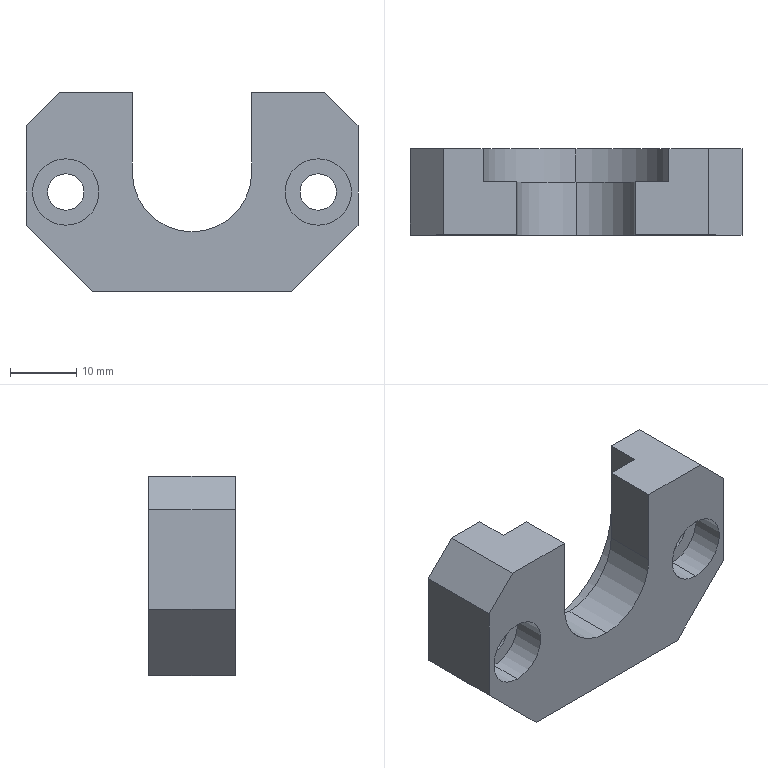Component | SolidWorks | F12529-M5112-1 | 1 solid | 30 faces | box 50 x 13 x 30 mm | volume 10744 mm3 | plane 18 | cylinder 12 | commonest cylinder face diameters 10 x4 5.5 x4 28 x2 18 x2
build123d program:
from build123d import *

# Parameters (mm, degrees)
SKETCH1_W                                            = 50
SKETCH1_H                                            = 30
BOSS_EXTRUDE1_DEPTH                                  = 13
CUT_EXTRUDE2_DEPTH                                   = 32.922
CUT_EXTRUDE3_DEPTH                                   = 5
M5_HEX_SOCKET_HEAD_CAP_SCREW_COUNTERBORE_D           = 5.5
M5_HEX_SOCKET_HEAD_CAP_SCREW_COUNTERBORE_CBORE_D     = 10
M5_HEX_SOCKET_HEAD_CAP_SCREW_COUNTERBORE_CBORE_DEPTH = 5
CHAMFER1_SIZE                                        = 5
CHAMFER2_SIZE                                        = 10


with BuildPart() as part:
    # Sketch1 → Boss-Extrude1 (new body)
    with BuildSketch(Plane(origin=(0, 0, 0), x_dir=(1, 0, 0), z_dir=(0, 1, 0))):
        Rectangle(SKETCH1_W, SKETCH1_H)
    extrude(amount=BOSS_EXTRUDE1_DEPTH)

    # Sketch2 → Cut-Extrude2 (cut, through all)
    with BuildSketch(Plane(origin=(0, 13, 0), x_dir=(1, 0, 0), z_dir=(0, 1, 0))):
        with BuildLine():
            Line((-9, 15), (9, 15))
            Line((9, 15), (9, 3))
            ThreePointArc((9, 3), (0, -6), (-9, 3))
            Line((-9, 3), (-9, 15))
        make_face()
    extrude(amount=-CUT_EXTRUDE2_DEPTH, mode=Mode.SUBTRACT)

    # Sketch3 → Cut-Extrude3 (cut)
    with BuildSketch(Plane(origin=(0, 13, 0), x_dir=(1, 0, 0), z_dir=(0, 1, 0))):
        with BuildLine():
            Line((-14, 15), (14, 15))
            Line((14, 15), (14, 3))
            ThreePointArc((14, 3), (0, -11), (-14, 3))
            Line((-14, 3), (-14, 15))
        make_face()
    extrude(amount=-CUT_EXTRUDE3_DEPTH, mode=Mode.SUBTRACT)

    # M5 Hex Socket Head Cap Screw Counterbore (through all)
    with Locations(Plane.XZ):
        with Locations((19, 0), (-19, 0)):
            CounterBoreHole(M5_HEX_SOCKET_HEAD_CAP_SCREW_COUNTERBORE_D / 2, M5_HEX_SOCKET_HEAD_CAP_SCREW_COUNTERBORE_CBORE_D / 2, M5_HEX_SOCKET_HEAD_CAP_SCREW_COUNTERBORE_CBORE_DEPTH)

    # Chamfer1
    chamfer1_edges = [part.edges().sort_by_distance(p)[0] for p in [
        (-25, 6.5, -15),
        (25, 6.5, -15),
    ]]
    chamfer(chamfer1_edges, length=CHAMFER1_SIZE)

    # Chamfer2
    chamfer2_edges = [part.edges().sort_by_distance(p)[0] for p in [
        (25, 6.5, 15),
        (-25, 6.5, 15),
    ]]
    chamfer(chamfer2_edges, length=CHAMFER2_SIZE)


solid = part.part

# Placed as in the assembly
solid = solid.moved(Location((0, 108, -3), (-180, 0, 180)))
STEP:
#1=CARTESIAN_POINT('',(-0.748,4.449,-0.315));
#2=VERTEX_POINT('',#1);
#3=CARTESIAN_POINT('',(-0.748,4.449,0.07874));
#4=VERTEX_POINT('',#3);
#5=CARTESIAN_POINT('',(-0.748,4.449,-0.1181));
#6=DIRECTION('',(-0.,-1.,-0.));
#7=DIRECTION('',(0.,0.,1.));
#8=AXIS2_PLACEMENT_3D('',#5,#6,#7);
#9=CIRCLE('',#8,0.1969);
#10=EDGE_CURVE('',#2,#4,#9,.T.);
#11=ORIENTED_EDGE('',*,*,#10,.F.);
#12=CARTESIAN_POINT('',(-0.748,4.252,-0.315));
#13=VERTEX_POINT('',#12);
#14=CARTESIAN_POINT('',(-0.748,4.252,-0.315));
#15=DIRECTION('',(-0.,-1.,-0.));
#16=VECTOR('',#15,39.37);
#17=LINE('',#14,#16);
#18=EDGE_CURVE('',#2,#13,#17,.T.);
#19=ORIENTED_EDGE('',*,*,#18,.T.);
#20=CARTESIAN_POINT('',(-0.748,4.252,0.07874));
#21=VERTEX_POINT('',#20);
#22=CARTESIAN_POINT('',(-0.748,4.252,-0.1181));
#23=DIRECTION('',(-0.,-1.,-0.));
#24=DIRECTION('',(0.,0.,1.));
#25=AXIS2_PLACEMENT_3D('',#22,#23,#24);
#26=CIRCLE('',#25,0.1969);
#27=EDGE_CURVE('',#13,#21,#26,.T.);
#28=ORIENTED_EDGE('',*,*,#27,.T.);
#29=CARTESIAN_POINT('',(-0.748,4.252,0.07874));
#30=DIRECTION('',(-0.,-1.,-0.));
#31=VECTOR('',#30,39.37);
#32=LINE('',#29,#31);
#33=EDGE_CURVE('',#4,#21,#32,.T.);
#34=ORIENTED_EDGE('',*,*,#33,.F.);
#35=EDGE_LOOP('',(#11,#19,#28,#34));
#36=FACE_OUTER_BOUND('',#35,.T.);
#37=CARTESIAN_POINT('',(-0.748,4.252,-0.1181));
#38=DIRECTION('',(-0.,-1.,-0.));
#39=DIRECTION('',(0.,0.,1.));
#40=AXIS2_PLACEMENT_3D('',#37,#38,#39);
#41=CYLINDRICAL_SURFACE('',#40,0.1969);
#42=ADVANCED_FACE('',(#36),#41,.F.);
#43=CARTESIAN_POINT('',(-0.748,4.764,-0.2264));
#44=VERTEX_POINT('',#43);
#45=CARTESIAN_POINT('',(-0.748,4.764,-0.009843));
#46=VERTEX_POINT('',#45);
#47=CARTESIAN_POINT('',(-0.748,4.764,-0.1181));
#48=DIRECTION('',(-0.,-1.,-0.));
#49=DIRECTION('',(0.,0.,1.));
#50=AXIS2_PLACEMENT_3D('',#47,#48,#49);
#51=CIRCLE('',#50,0.1083);
#52=EDGE_CURVE('',#44,#46,#51,.T.);
#53=ORIENTED_EDGE('',*,*,#52,.F.);
#54=CARTESIAN_POINT('',(-0.748,4.449,-0.2264));
#55=VERTEX_POINT('',#54);
#56=CARTESIAN_POINT('',(-0.748,4.252,-0.2264));
#57=DIRECTION('',(-0.,-1.,-0.));
#58=VECTOR('',#57,39.37);
#59=LINE('',#56,#58);
#60=EDGE_CURVE('',#44,#55,#59,.T.);
#61=ORIENTED_EDGE('',*,*,#60,.T.);
#62=CARTESIAN_POINT('',(-0.748,4.449,-0.009843));
#63=VERTEX_POINT('',#62);
#64=CARTESIAN_POINT('',(-0.748,4.449,-0.1181));
#65=DIRECTION('',(-0.,-1.,-0.));
#66=DIRECTION('',(0.,0.,1.));
#67=AXIS2_PLACEMENT_3D('',#64,#65,#66);
#68=CIRCLE('',#67,0.1083);
#69=EDGE_CURVE('',#55,#63,#68,.T.);
#70=ORIENTED_EDGE('',*,*,#69,.T.);
#71=CARTESIAN_POINT('',(-0.748,4.252,-0.009843));
#72=DIRECTION('',(-0.,-1.,-0.));
#73=VECTOR('',#72,39.37);
#74=LINE('',#71,#73);
#75=EDGE_CURVE('',#46,#63,#74,.T.);
#76=ORIENTED_EDGE('',*,*,#75,.F.);
#77=EDGE_LOOP('',(#53,#61,#70,#76));
#78=FACE_OUTER_BOUND('',#77,.T.);
#79=CARTESIAN_POINT('',(-0.748,4.252,-0.1181));
#80=DIRECTION('',(-0.,-1.,-0.));
#81=DIRECTION('',(0.,0.,1.));
#82=AXIS2_PLACEMENT_3D('',#79,#80,#81);
#83=CYLINDRICAL_SURFACE('',#82,0.1083);
#84=ADVANCED_FACE('',(#78),#83,.F.);
#85=CARTESIAN_POINT('',(0.748,4.449,-0.315));
#86=VERTEX_POINT('',#85);
#87=CARTESIAN_POINT('',(0.748,4.449,0.07874));
#88=VERTEX_POINT('',#87);
#89=CARTESIAN_POINT('',(0.748,4.449,-0.1181));
#90=DIRECTION('',(-0.,-1.,-0.));
#91=DIRECTION('',(0.,0.,1.));
#92=AXIS2_PLACEMENT_3D('',#89,#90,#91);
#93=CIRCLE('',#92,0.1969);
#94=EDGE_CURVE('',#86,#88,#93,.T.);
#95=ORIENTED_EDGE('',*,*,#94,.F.);
#96=CARTESIAN_POINT('',(0.748,4.252,-0.315));
#97=VERTEX_POINT('',#96);
#98=CARTESIAN_POINT('',(0.748,4.252,-0.315));
#99=DIRECTION('',(-0.,-1.,-0.));
#100=VECTOR('',#99,39.37);
#101=LINE('',#98,#100);
#102=EDGE_CURVE('',#86,#97,#101,.T.);
#103=ORIENTED_EDGE('',*,*,#102,.T.);
#104=CARTESIAN_POINT('',(0.748,4.252,0.07874));
#105=VERTEX_POINT('',#104);
#106=CARTESIAN_POINT('',(0.748,4.252,-0.1181));
#107=DIRECTION('',(-0.,-1.,-0.));
#108=DIRECTION('',(0.,0.,1.));
#109=AXIS2_PLACEMENT_3D('',#106,#107,#108);
#110=CIRCLE('',#109,0.1969);
#111=EDGE_CURVE('',#97,#105,#110,.T.);
#112=ORIENTED_EDGE('',*,*,#111,.T.);
#113=CARTESIAN_POINT('',(0.748,4.252,0.07874));
#114=DIRECTION('',(-0.,-1.,-0.));
#115=VECTOR('',#114,39.37);
#116=LINE('',#113,#115);
#117=EDGE_CURVE('',#88,#105,#116,.T.);
#118=ORIENTED_EDGE('',*,*,#117,.F.);
#119=EDGE_LOOP('',(#95,#103,#112,#118));
#120=FACE_OUTER_BOUND('',#119,.T.);
#121=CARTESIAN_POINT('',(0.748,4.252,-0.1181));
#122=DIRECTION('',(-0.,-1.,-0.));
#123=DIRECTION('',(0.,0.,1.));
#124=AXIS2_PLACEMENT_3D('',#121,#122,#123);
#125=CYLINDRICAL_SURFACE('',#124,0.1969);
#126=ADVANCED_FACE('',(#120),#125,.F.);
#127=CARTESIAN_POINT('',(0.748,4.764,-0.2264));
#128=VERTEX_POINT('',#127);
#129=CARTESIAN_POINT('',(0.748,4.764,-0.009843));
#130=VERTEX_POINT('',#129);
#131=CARTESIAN_POINT('',(0.748,4.764,-0.1181));
#132=DIRECTION('',(-0.,-1.,-0.));
#133=DIRECTION('',(0.,0.,1.));
#134=AXIS2_PLACEMENT_3D('',#131,#132,#133);
#135=CIRCLE('',#134,0.1083);
#136=EDGE_CURVE('',#128,#130,#135,.T.);
#137=ORIENTED_EDGE('',*,*,#136,.F.);
#138=CARTESIAN_POINT('',(0.748,4.449,-0.2264));
#139=VERTEX_POINT('',#138);
#140=CARTESIAN_POINT('',(0.748,4.252,-0.2264));
#141=DIRECTION('',(-0.,-1.,-0.));
#142=VECTOR('',#141,39.37);
#143=LINE('',#140,#142);
#144=EDGE_CURVE('',#128,#139,#143,.T.);
#145=ORIENTED_EDGE('',*,*,#144,.T.);
#146=CARTESIAN_POINT('',(0.748,4.449,-0.009843));
#147=VERTEX_POINT('',#146);
#148=CARTESIAN_POINT('',(0.748,4.449,-0.1181));
#149=DIRECTION('',(-0.,-1.,-0.));
#150=DIRECTION('',(0.,0.,1.));
#151=AXIS2_PLACEMENT_3D('',#148,#149,#150);
#152=CIRCLE('',#151,0.1083);
#153=EDGE_CURVE('',#139,#147,#152,.T.);
#154=ORIENTED_EDGE('',*,*,#153,.T.);
#155=CARTESIAN_POINT('',(0.748,4.252,-0.009843));
#156=DIRECTION('',(-0.,-1.,-0.));
#157=VECTOR('',#156,39.37);
#158=LINE('',#155,#157);
#159=EDGE_CURVE('',#130,#147,#158,.T.);
#160=ORIENTED_EDGE('',*,*,#159,.F.);
#161=EDGE_LOOP('',(#137,#145,#154,#160));
#162=FACE_OUTER_BOUND('',#161,.T.);
#163=CARTESIAN_POINT('',(0.748,4.252,-0.1181));
#164=DIRECTION('',(-0.,-1.,-0.));
#165=DIRECTION('',(0.,0.,1.));
#166=AXIS2_PLACEMENT_3D('',#163,#164,#165);
#167=CYLINDRICAL_SURFACE('',#166,0.1083);
#168=ADVANCED_FACE('',(#162),#167,.F.);
#169=CARTESIAN_POINT('',(0.,4.567,-0.5512));
#170=VERTEX_POINT('',#169);
#171=CARTESIAN_POINT('',(-0.5512,4.567,0.));
#172=VERTEX_POINT('',#171);
#173=CARTESIAN_POINT('',(0.,4.567,0.));
#174=DIRECTION('',(0.,1.,0.));
#175=DIRECTION('',(-0.,0.,1.));
#176=AXIS2_PLACEMENT_3D('',#173,#174,#175);
#177=CIRCLE('',#176,0.5512);
#178=EDGE_CURVE('',#170,#172,#177,.T.);
#179=ORIENTED_EDGE('',*,*,#178,.F.);
#180=CARTESIAN_POINT('',(0.,4.764,-0.5512));
#181=VERTEX_POINT('',#180);
#182=CARTESIAN_POINT('',(0.,4.567,-0.5512));
#183=DIRECTION('',(0.,1.,0.));
#184=VECTOR('',#183,39.37);
#185=LINE('',#182,#184);
#186=EDGE_CURVE('',#170,#181,#185,.T.);
#187=ORIENTED_EDGE('',*,*,#186,.T.);
#188=CARTESIAN_POINT('',(-0.5512,4.764,0.));
#189=VERTEX_POINT('',#188);
#190=CARTESIAN_POINT('',(0.,4.764,0.));
#191=DIRECTION('',(0.,1.,0.));
#192=DIRECTION('',(-0.,0.,1.));
#193=AXIS2_PLACEMENT_3D('',#190,#191,#192);
#194=CIRCLE('',#193,0.5512);
#195=EDGE_CURVE('',#181,#189,#194,.T.);
#196=ORIENTED_EDGE('',*,*,#195,.T.);
#197=CARTESIAN_POINT('',(-0.5512,4.567,0.));
#198=DIRECTION('',(0.,1.,0.));
#199=VECTOR('',#198,39.37);
#200=LINE('',#197,#199);
#201=EDGE_CURVE('',#172,#189,#200,.T.);
#202=ORIENTED_EDGE('',*,*,#201,.F.);
#203=EDGE_LOOP('',(#179,#187,#196,#202));
#204=FACE_OUTER_BOUND('',#203,.T.);
#205=CARTESIAN_POINT('',(0.,4.567,0.));
#206=DIRECTION('',(0.,1.,0.));
#207=DIRECTION('',(0.,0.,-1.));
#208=AXIS2_PLACEMENT_3D('',#205,#206,#207);
#209=CYLINDRICAL_SURFACE('',#208,0.5512);
#210=ADVANCED_FACE('',(#204),#209,.F.);
#211=CARTESIAN_POINT('',(0.,4.252,-0.3543));
#212=VERTEX_POINT('',#211);
#213=CARTESIAN_POINT('',(-0.3543,4.252,0.));
#214=VERTEX_POINT('',#213);
#215=CARTESIAN_POINT('',(0.,4.252,0.));
#216=DIRECTION('',(0.,1.,0.));
#217=DIRECTION('',(-0.,0.,1.));
#218=AXIS2_PLACEMENT_3D('',#215,#216,#217);
#219=CIRCLE('',#218,0.3543);
#220=EDGE_CURVE('',#212,#214,#219,.T.);
#221=ORIENTED_EDGE('',*,*,#220,.F.);
#222=CARTESIAN_POINT('',(0.,4.567,-0.3543));
#223=VERTEX_POINT('',#222);
#224=CARTESIAN_POINT('',(0.,4.252,-0.3543));
#225=DIRECTION('',(0.,1.,0.));
#226=VECTOR('',#225,39.37);
#227=LINE('',#224,#226);
#228=EDGE_CURVE('',#212,#223,#227,.T.);
#229=ORIENTED_EDGE('',*,*,#228,.T.);
#230=CARTESIAN_POINT('',(-0.3543,4.567,0.));
#231=VERTEX_POINT('',#230);
#232=CARTESIAN_POINT('',(0.,4.567,0.));
#233=DIRECTION('',(0.,1.,0.));
#234=DIRECTION('',(-0.,0.,1.));
#235=AXIS2_PLACEMENT_3D('',#232,#233,#234);
#236=CIRCLE('',#235,0.3543);
#237=EDGE_CURVE('',#223,#231,#236,.T.);
#238=ORIENTED_EDGE('',*,*,#237,.T.);
#239=CARTESIAN_POINT('',(-0.3543,4.252,0.));
#240=DIRECTION('',(0.,1.,0.));
#241=VECTOR('',#240,39.37);
#242=LINE('',#239,#241);
#243=EDGE_CURVE('',#214,#231,#242,.T.);
#244=ORIENTED_EDGE('',*,*,#243,.F.);
#245=EDGE_LOOP('',(#221,#229,#238,#244));
#246=FACE_OUTER_BOUND('',#245,.T.);
#247=CARTESIAN_POINT('',(0.,4.252,0.));
#248=DIRECTION('',(0.,1.,0.));
#249=DIRECTION('',(0.,0.,-1.));
#250=AXIS2_PLACEMENT_3D('',#247,#248,#249);
#251=CYLINDRICAL_SURFACE('',#250,0.3543);
#252=ADVANCED_FACE('',(#246),#251,.F.);
#253=CARTESIAN_POINT('',(0.3543,4.252,0.4724));
#254=VERTEX_POINT('',#253);
#255=CARTESIAN_POINT('',(0.7874,4.252,0.4724));
#256=VERTEX_POINT('',#255);
#257=CARTESIAN_POINT('',(0.9843,4.252,0.4724));
#258=DIRECTION('',(1.,-0.,0.));
#259=VECTOR('',#258,39.37);
#260=LINE('',#257,#259);
#261=EDGE_CURVE('',#254,#256,#260,.T.);
#262=ORIENTED_EDGE('',*,*,#261,.T.);
#263=CARTESIAN_POINT('',(0.7874,4.764,0.4724));
#264=VERTEX_POINT('',#263);
#265=CARTESIAN_POINT('',(0.7874,4.764,0.4724));
#266=DIRECTION('',(0.,1.,0.));
#267=VECTOR('',#266,39.37);
#268=LINE('',#265,#267);
#269=EDGE_CURVE('',#256,#264,#268,.T.);
#270=ORIENTED_EDGE('',*,*,#269,.T.);
#271=CARTESIAN_POINT('',(0.5512,4.764,0.4724));
#272=VERTEX_POINT('',#271);
#273=CARTESIAN_POINT('',(0.9843,4.764,0.4724));
#274=DIRECTION('',(1.,-0.,0.));
#275=VECTOR('',#274,39.37);
#276=LINE('',#273,#275);
#277=EDGE_CURVE('',#272,#264,#276,.T.);
#278=ORIENTED_EDGE('',*,*,#277,.F.);
#279=CARTESIAN_POINT('',(0.5512,4.567,0.4724));
#280=VERTEX_POINT('',#279);
#281=CARTESIAN_POINT('',(0.5512,4.567,0.4724));
#282=DIRECTION('',(0.,1.,0.));
#283=VECTOR('',#282,39.37);
#284=LINE('',#281,#283);
#285=EDGE_CURVE('',#280,#272,#284,.T.);
#286=ORIENTED_EDGE('',*,*,#285,.F.);
#287=CARTESIAN_POINT('',(0.3543,4.567,0.4724));
#288=VERTEX_POINT('',#287);
#289=CARTESIAN_POINT('',(0.5512,4.567,0.4724));
#290=DIRECTION('',(1.,-0.,0.));
#291=VECTOR('',#290,39.37);
#292=LINE('',#289,#291);
#293=EDGE_CURVE('',#288,#280,#292,.T.);
#294=ORIENTED_EDGE('',*,*,#293,.F.);
#295=CARTESIAN_POINT('',(0.3543,4.252,0.4724));
#296=DIRECTION('',(0.,1.,0.));
#297=VECTOR('',#296,39.37);
#298=LINE('',#295,#297);
#299=EDGE_CURVE('',#254,#288,#298,.T.);
#300=ORIENTED_EDGE('',*,*,#299,.F.);
#301=EDGE_LOOP('',(#262,#270,#278,#286,#294,#300));
#302=FACE_OUTER_BOUND('',#301,.T.);
#303=CARTESIAN_POINT('',(0.9843,4.764,0.4724));
#304=DIRECTION('',(0.,0.,-1.));
#305=DIRECTION('',(-1.,0.,-0.));
#306=AXIS2_PLACEMENT_3D('',#303,#304,#305);
#307=PLANE('',#306);
#308=ADVANCED_FACE('',(#302),#307,.F.);
#309=CARTESIAN_POINT('',(0.9843,4.252,0.2756));
#310=VERTEX_POINT('',#309);
#311=CARTESIAN_POINT('',(0.9843,4.252,-0.315));
#312=VERTEX_POINT('',#311);
#313=CARTESIAN_POINT('',(0.9843,4.252,0.4724));
#314=DIRECTION('',(-0.,0.,-1.));
#315=VECTOR('',#314,39.37);
#316=LINE('',#313,#315);
#317=EDGE_CURVE('',#310,#312,#316,.T.);
#318=ORIENTED_EDGE('',*,*,#317,.T.);
#319=CARTESIAN_POINT('',(0.9843,4.764,-0.315));
#320=VERTEX_POINT('',#319);
#321=CARTESIAN_POINT('',(0.9843,4.764,-0.315));
#322=DIRECTION('',(0.,1.,0.));
#323=VECTOR('',#322,39.37);
#324=LINE('',#321,#323);
#325=EDGE_CURVE('',#312,#320,#324,.T.);
#326=ORIENTED_EDGE('',*,*,#325,.T.);
#327=CARTESIAN_POINT('',(0.9843,4.764,0.2756));
#328=VERTEX_POINT('',#327);
#329=CARTESIAN_POINT('',(0.9843,4.764,0.4724));
#330=DIRECTION('',(-0.,0.,-1.));
#331=VECTOR('',#330,39.37);
#332=LINE('',#329,#331);
#333=EDGE_CURVE('',#328,#320,#332,.T.);
#334=ORIENTED_EDGE('',*,*,#333,.F.);
#335=CARTESIAN_POINT('',(0.9843,4.764,0.2756));
#336=DIRECTION('',(-0.,-1.,-0.));
#337=VECTOR('',#336,39.37);
#338=LINE('',#335,#337);
#339=EDGE_CURVE('',#328,#310,#338,.T.);
#340=ORIENTED_EDGE('',*,*,#339,.T.);
#341=EDGE_LOOP('',(#318,#326,#334,#340));
#342=FACE_OUTER_BOUND('',#341,.T.);
#343=CARTESIAN_POINT('',(0.9843,4.764,0.4724));
#344=DIRECTION('',(-1.,0.,0.));
#345=DIRECTION('',(0.,-0.,1.));
#346=AXIS2_PLACEMENT_3D('',#343,#344,#345);
#347=PLANE('',#346);
#348=ADVANCED_FACE('',(#342),#347,.F.);
#349=CARTESIAN_POINT('',(0.5906,4.252,-0.7087));
#350=VERTEX_POINT('',#349);
#351=CARTESIAN_POINT('',(-0.5906,4.252,-0.7087));
#352=VERTEX_POINT('',#351);
#353=CARTESIAN_POINT('',(0.9843,4.252,-0.7087));
#354=DIRECTION('',(-1.,0.,-0.));
#355=VECTOR('',#354,39.37);
#356=LINE('',#353,#355);
#357=EDGE_CURVE('',#350,#352,#356,.T.);
#358=ORIENTED_EDGE('',*,*,#357,.T.);
#359=CARTESIAN_POINT('',(-0.5906,4.764,-0.7087));
#360=VERTEX_POINT('',#359);
#361=CARTESIAN_POINT('',(-0.5906,4.764,-0.7087));
#362=DIRECTION('',(0.,1.,0.));
#363=VECTOR('',#362,39.37);
#364=LINE('',#361,#363);
#365=EDGE_CURVE('',#352,#360,#364,.T.);
#366=ORIENTED_EDGE('',*,*,#365,.T.);
#367=CARTESIAN_POINT('',(0.5906,4.764,-0.7087));
#368=VERTEX_POINT('',#367);
#369=CARTESIAN_POINT('',(0.9843,4.764,-0.7087));
#370=DIRECTION('',(-1.,0.,-0.));
#371=VECTOR('',#370,39.37);
#372=LINE('',#369,#371);
#373=EDGE_CURVE('',#368,#360,#372,.T.);
#374=ORIENTED_EDGE('',*,*,#373,.F.);
#375=CARTESIAN_POINT('',(0.5906,4.764,-0.7087));
#376=DIRECTION('',(-0.,-1.,-0.));
#377=VECTOR('',#376,39.37);
#378=LINE('',#375,#377);
#379=EDGE_CURVE('',#368,#350,#378,.T.);
#380=ORIENTED_EDGE('',*,*,#379,.T.);
#381=EDGE_LOOP('',(#358,#366,#374,#380));
#382=FACE_OUTER_BOUND('',#381,.T.);
#383=CARTESIAN_POINT('',(0.9843,4.764,-0.7087));
#384=DIRECTION('',(-0.,-0.,1.));
#385=DIRECTION('',(1.,-0.,0.));
#386=AXIS2_PLACEMENT_3D('',#383,#384,#385);
#387=PLANE('',#386);
#388=ADVANCED_FACE('',(#382),#387,.F.);
#389=CARTESIAN_POINT('',(-0.9843,4.764,-0.315));
#390=VERTEX_POINT('',#389);
#391=CARTESIAN_POINT('',(-0.9843,4.764,0.2756));
#392=VERTEX_POINT('',#391);
#393=CARTESIAN_POINT('',(-0.9843,4.764,0.4724));
#394=DIRECTION('',(0.,-0.,1.));
#395=VECTOR('',#394,39.37);
#396=LINE('',#393,#395);
#397=EDGE_CURVE('',#390,#392,#396,.T.);
#398=ORIENTED_EDGE('',*,*,#397,.F.);
#399=CARTESIAN_POINT('',(-0.9843,4.252,-0.315));
#400=VERTEX_POINT('',#399);
#401=CARTESIAN_POINT('',(-0.9843,4.764,-0.315));
#402=DIRECTION('',(-0.,-1.,-0.));
#403=VECTOR('',#402,39.37);
#404=LINE('',#401,#403);
#405=EDGE_CURVE('',#390,#400,#404,.T.);
#406=ORIENTED_EDGE('',*,*,#405,.T.);
#407=CARTESIAN_POINT('',(-0.9843,4.252,0.2756));
#408=VERTEX_POINT('',#407);
#409=CARTESIAN_POINT('',(-0.9843,4.252,0.4724));
#410=DIRECTION('',(0.,-0.,1.));
#411=VECTOR('',#410,39.37);
#412=LINE('',#409,#411);
#413=EDGE_CURVE('',#400,#408,#412,.T.);
#414=ORIENTED_EDGE('',*,*,#413,.T.);
#415=CARTESIAN_POINT('',(-0.9843,4.764,0.2756));
#416=DIRECTION('',(0.,1.,0.));
#417=VECTOR('',#416,39.37);
#418=LINE('',#415,#417);
#419=EDGE_CURVE('',#408,#392,#418,.T.);
#420=ORIENTED_EDGE('',*,*,#419,.T.);
#421=EDGE_LOOP('',(#398,#406,#414,#420));
#422=FACE_OUTER_BOUND('',#421,.T.);
#423=CARTESIAN_POINT('',(-0.9843,4.764,0.4724));
#424=DIRECTION('',(1.,-0.,-0.));
#425=DIRECTION('',(-0.,0.,-1.));
#426=AXIS2_PLACEMENT_3D('',#423,#424,#425);
#427=PLANE('',#426);
#428=ADVANCED_FACE('',(#422),#427,.F.);
#429=CARTESIAN_POINT('',(-0.7874,4.764,0.4724));
#430=VERTEX_POINT('',#429);
#431=CARTESIAN_POINT('',(-0.5512,4.764,0.4724));
#432=VERTEX_POINT('',#431);
#433=CARTESIAN_POINT('',(0.9843,4.764,0.4724));
#434=DIRECTION('',(1.,-0.,0.));
#435=VECTOR('',#434,39.37);
#436=LINE('',#433,#435);
#437=EDGE_CURVE('',#430,#432,#436,.T.);
#438=ORIENTED_EDGE('',*,*,#437,.F.);
#439=CARTESIAN_POINT('',(-0.7874,4.252,0.4724));
#440=VERTEX_POINT('',#439);
#441=CARTESIAN_POINT('',(-0.7874,4.764,0.4724));
#442=DIRECTION('',(-0.,-1.,-0.));
#443=VECTOR('',#442,39.37);
#444=LINE('',#441,#443);
#445=EDGE_CURVE('',#430,#440,#444,.T.);
#446=ORIENTED_EDGE('',*,*,#445,.T.);
#447=CARTESIAN_POINT('',(-0.3543,4.252,0.4724));
#448=VERTEX_POINT('',#447);
#449=CARTESIAN_POINT('',(0.9843,4.252,0.4724));
#450=DIRECTION('',(1.,-0.,0.));
#451=VECTOR('',#450,39.37);
#452=LINE('',#449,#451);
#453=EDGE_CURVE('',#440,#448,#452,.T.);
#454=ORIENTED_EDGE('',*,*,#453,.T.);
#455=CARTESIAN_POINT('',(-0.3543,4.567,0.4724));
#456=VERTEX_POINT('',#455);
#457=CARTESIAN_POINT('',(-0.3543,4.252,0.4724));
#458=DIRECTION('',(0.,1.,0.));
#459=VECTOR('',#458,39.37);
#460=LINE('',#457,#459);
#461=EDGE_CURVE('',#448,#456,#460,.T.);
#462=ORIENTED_EDGE('',*,*,#461,.T.);
#463=CARTESIAN_POINT('',(-0.5512,4.567,0.4724));
#464=VERTEX_POINT('',#463);
#465=CARTESIAN_POINT('',(0.5512,4.567,0.4724));
#466=DIRECTION('',(1.,-0.,0.));
#467=VECTOR('',#466,39.37);
#468=LINE('',#465,#467);
#469=EDGE_CURVE('',#464,#456,#468,.T.);
#470=ORIENTED_EDGE('',*,*,#469,.F.);
#471=CARTESIAN_POINT('',(-0.5512,4.567,0.4724));
#472=DIRECTION('',(0.,1.,0.));
#473=VECTOR('',#472,39.37);
#474=LINE('',#471,#473);
#475=EDGE_CURVE('',#464,#432,#474,.T.);
#476=ORIENTED_EDGE('',*,*,#475,.T.);
#477=EDGE_LOOP('',(#438,#446,#454,#462,#470,#476));
#478=FACE_OUTER_BOUND('',#477,.T.);
#479=CARTESIAN_POINT('',(0.9843,4.764,0.4724));
#480=DIRECTION('',(0.,0.,-1.));
#481=DIRECTION('',(-1.,0.,-0.));
#482=AXIS2_PLACEMENT_3D('',#479,#480,#481);
#483=PLANE('',#482);
#484=ADVANCED_FACE('',(#478),#483,.F.);
#485=CARTESIAN_POINT('',(-0.748,4.764,-0.1181));
#486=DIRECTION('',(-0.,-1.,-0.));
#487=DIRECTION('',(0.,0.,1.));
#488=AXIS2_PLACEMENT_3D('',#485,#486,#487);
#489=CIRCLE('',#488,0.1083);
#490=EDGE_CURVE('',#46,#44,#489,.T.);
#491=ORIENTED_EDGE('',*,*,#490,.T.);
#492=ORIENTED_EDGE('',*,*,#52,.T.);
#493=EDGE_LOOP('',(#491,#492));
#494=FACE_BOUND('',#493,.T.);
#495=CARTESIAN_POINT('',(0.748,4.764,-0.1181));
#496=DIRECTION('',(-0.,-1.,-0.));
#497=DIRECTION('',(0.,0.,1.));
#498=AXIS2_PLACEMENT_3D('',#495,#496,#497);
#499=CIRCLE('',#498,0.1083);
#500=EDGE_CURVE('',#130,#128,#499,.T.);
#501=ORIENTED_EDGE('',*,*,#500,.T.);
#502=ORIENTED_EDGE('',*,*,#136,.T.);
#503=EDGE_LOOP('',(#501,#502));
#504=FACE_BOUND('',#503,.T.);
#505=ORIENTED_EDGE('',*,*,#373,.T.);
#506=CARTESIAN_POINT('',(0.1969,4.764,-1.496));
#507=DIRECTION('',(-0.7071,-0.,0.7071));
#508=VECTOR('',#507,39.37);
#509=LINE('',#506,#508);
#510=EDGE_CURVE('',#360,#390,#509,.T.);
#511=ORIENTED_EDGE('',*,*,#510,.T.);
#512=ORIENTED_EDGE('',*,*,#397,.T.);
#513=CARTESIAN_POINT('',(-0.4921,4.764,0.7677));
#514=DIRECTION('',(0.7071,-0.,0.7071));
#515=VECTOR('',#514,39.37);
#516=LINE('',#513,#515);
#517=EDGE_CURVE('',#392,#430,#516,.T.);
#518=ORIENTED_EDGE('',*,*,#517,.T.);
#519=ORIENTED_EDGE('',*,*,#437,.T.);
#520=CARTESIAN_POINT('',(-0.5512,4.764,0.4724));
#521=DIRECTION('',(-0.,-0.,1.));
#522=VECTOR('',#521,39.37);
#523=LINE('',#520,#522);
#524=EDGE_CURVE('',#189,#432,#523,.T.);
#525=ORIENTED_EDGE('',*,*,#524,.F.);
#526=ORIENTED_EDGE('',*,*,#195,.F.);
#527=CARTESIAN_POINT('',(0.5512,4.764,0.));
#528=VERTEX_POINT('',#527);
#529=CARTESIAN_POINT('',(0.,4.764,0.));
#530=DIRECTION('',(0.,1.,0.));
#531=DIRECTION('',(-0.,0.,1.));
#532=AXIS2_PLACEMENT_3D('',#529,#530,#531);
#533=CIRCLE('',#532,0.5512);
#534=EDGE_CURVE('',#528,#181,#533,.T.);
#535=ORIENTED_EDGE('',*,*,#534,.F.);
#536=CARTESIAN_POINT('',(0.5512,4.764,0.4724));
#537=DIRECTION('',(-0.,0.,-1.));
#538=VECTOR('',#537,39.37);
#539=LINE('',#536,#538);
#540=EDGE_CURVE('',#272,#528,#539,.T.);
#541=ORIENTED_EDGE('',*,*,#540,.F.);
#542=ORIENTED_EDGE('',*,*,#277,.T.);
#543=CARTESIAN_POINT('',(1.476,4.764,-0.2165));
#544=DIRECTION('',(0.7071,0.,-0.7071));
#545=VECTOR('',#544,39.37);
#546=LINE('',#543,#545);
#547=EDGE_CURVE('',#264,#328,#546,.T.);
#548=ORIENTED_EDGE('',*,*,#547,.T.);
#549=ORIENTED_EDGE('',*,*,#333,.T.);
#550=CARTESIAN_POINT('',(0.7874,4.764,-0.5118));
#551=DIRECTION('',(-0.7071,0.,-0.7071));
#552=VECTOR('',#551,39.37);
#553=LINE('',#550,#552);
#554=EDGE_CURVE('',#320,#368,#553,.T.);
#555=ORIENTED_EDGE('',*,*,#554,.T.);
#556=EDGE_LOOP('',(#505,#511,#512,#518,#519,#525,#526,#535,#541,#542,#548,#549,#555));
#557=FACE_OUTER_BOUND('',#556,.T.);
#558=CARTESIAN_POINT('',(0.9843,4.764,-0.7087));
#559=DIRECTION('',(0.,1.,0.));
#560=DIRECTION('',(0.,0.,-1.));
#561=AXIS2_PLACEMENT_3D('',#558,#559,#560);
#562=PLANE('',#561);
#563=ADVANCED_FACE('',(#494,#504,#557),#562,.T.);
#564=CARTESIAN_POINT('',(-0.748,4.252,-0.1181));
#565=DIRECTION('',(-0.,-1.,-0.));
#566=DIRECTION('',(0.,0.,1.));
#567=AXIS2_PLACEMENT_3D('',#564,#565,#566);
#568=CIRCLE('',#567,0.1969);
#569=EDGE_CURVE('',#21,#13,#568,.T.);
#570=ORIENTED_EDGE('',*,*,#569,.F.);
#571=ORIENTED_EDGE('',*,*,#27,.F.);
#572=EDGE_LOOP('',(#570,#571));
#573=FACE_BOUND('',#572,.T.);
#574=CARTESIAN_POINT('',(0.748,4.252,-0.1181));
#575=DIRECTION('',(-0.,-1.,-0.));
#576=DIRECTION('',(0.,0.,1.));
#577=AXIS2_PLACEMENT_3D('',#574,#575,#576);
#578=CIRCLE('',#577,0.1969);
#579=EDGE_CURVE('',#105,#97,#578,.T.);
#580=ORIENTED_EDGE('',*,*,#579,.F.);
#581=ORIENTED_EDGE('',*,*,#111,.F.);
#582=EDGE_LOOP('',(#580,#581));
#583=FACE_BOUND('',#582,.T.);
#584=ORIENTED_EDGE('',*,*,#413,.F.);
#585=CARTESIAN_POINT('',(-0.9843,4.252,-0.315));
#586=DIRECTION('',(0.7071,0.,-0.7071));
#587=VECTOR('',#586,39.37);
#588=LINE('',#585,#587);
#589=EDGE_CURVE('',#400,#352,#588,.T.);
#590=ORIENTED_EDGE('',*,*,#589,.T.);
#591=ORIENTED_EDGE('',*,*,#357,.F.);
#592=CARTESIAN_POINT('',(0.5906,4.252,-0.7087));
#593=DIRECTION('',(0.7071,-0.,0.7071));
#594=VECTOR('',#593,39.37);
#595=LINE('',#592,#594);
#596=EDGE_CURVE('',#350,#312,#595,.T.);
#597=ORIENTED_EDGE('',*,*,#596,.T.);
#598=ORIENTED_EDGE('',*,*,#317,.F.);
#599=CARTESIAN_POINT('',(0.9843,4.252,0.2756));
#600=DIRECTION('',(-0.7071,-0.,0.7071));
#601=VECTOR('',#600,39.37);
#602=LINE('',#599,#601);
#603=EDGE_CURVE('',#310,#256,#602,.T.);
#604=ORIENTED_EDGE('',*,*,#603,.T.);
#605=ORIENTED_EDGE('',*,*,#261,.F.);
#606=CARTESIAN_POINT('',(0.3543,4.252,0.));
#607=VERTEX_POINT('',#606);
#608=CARTESIAN_POINT('',(0.3543,4.252,0.4724));
#609=DIRECTION('',(0.,0.,-1.));
#610=VECTOR('',#609,39.37);
#611=LINE('',#608,#610);
#612=EDGE_CURVE('',#254,#607,#611,.T.);
#613=ORIENTED_EDGE('',*,*,#612,.T.);
#614=CARTESIAN_POINT('',(0.,4.252,0.));
#615=DIRECTION('',(0.,1.,0.));
#616=DIRECTION('',(-0.,0.,1.));
#617=AXIS2_PLACEMENT_3D('',#614,#615,#616);
#618=CIRCLE('',#617,0.3543);
#619=EDGE_CURVE('',#607,#212,#618,.T.);
#620=ORIENTED_EDGE('',*,*,#619,.T.);
#621=ORIENTED_EDGE('',*,*,#220,.T.);
#622=CARTESIAN_POINT('',(-0.3543,4.252,0.4724));
#623=DIRECTION('',(-0.,-0.,1.));
#624=VECTOR('',#623,39.37);
#625=LINE('',#622,#624);
#626=EDGE_CURVE('',#214,#448,#625,.T.);
#627=ORIENTED_EDGE('',*,*,#626,.T.);
#628=ORIENTED_EDGE('',*,*,#453,.F.);
#629=CARTESIAN_POINT('',(-0.7874,4.252,0.4724));
#630=DIRECTION('',(-0.7071,0.,-0.7071));
#631=VECTOR('',#630,39.37);
#632=LINE('',#629,#631);
#633=EDGE_CURVE('',#440,#408,#632,.T.);
#634=ORIENTED_EDGE('',*,*,#633,.T.);
#635=EDGE_LOOP('',(#584,#590,#591,#597,#598,#604,#605,#613,#620,#621,#627,#628,#634));
#636=FACE_OUTER_BOUND('',#635,.T.);
#637=CARTESIAN_POINT('',(0.9843,4.252,-0.7087));
#638=DIRECTION('',(0.,1.,0.));
#639=DIRECTION('',(0.,0.,-1.));
#640=AXIS2_PLACEMENT_3D('',#637,#638,#639);
#641=PLANE('',#640);
#642=ADVANCED_FACE('',(#573,#583,#636),#641,.F.);
#643=ORIENTED_EDGE('',*,*,#299,.T.);
#644=CARTESIAN_POINT('',(0.3543,4.567,0.));
#645=VERTEX_POINT('',#644);
#646=CARTESIAN_POINT('',(0.3543,4.567,0.4724));
#647=DIRECTION('',(0.,0.,-1.));
#648=VECTOR('',#647,39.37);
#649=LINE('',#646,#648);
#650=EDGE_CURVE('',#288,#645,#649,.T.);
#651=ORIENTED_EDGE('',*,*,#650,.T.);
#652=CARTESIAN_POINT('',(0.3543,4.252,0.));
#653=DIRECTION('',(0.,1.,0.));
#654=VECTOR('',#653,39.37);
#655=LINE('',#652,#654);
#656=EDGE_CURVE('',#607,#645,#655,.T.);
#657=ORIENTED_EDGE('',*,*,#656,.F.);
#658=ORIENTED_EDGE('',*,*,#612,.F.);
#659=EDGE_LOOP('',(#643,#651,#657,#658));
#660=FACE_OUTER_BOUND('',#659,.T.);
#661=CARTESIAN_POINT('',(0.3543,4.252,0.4724));
#662=DIRECTION('',(1.,-0.,0.));
#663=DIRECTION('',(0.,0.,-1.));
#664=AXIS2_PLACEMENT_3D('',#661,#662,#663);
#665=PLANE('',#664);
#666=ADVANCED_FACE('',(#660),#665,.F.);
#667=ORIENTED_EDGE('',*,*,#243,.T.);
#668=CARTESIAN_POINT('',(-0.3543,4.567,0.4724));
#669=DIRECTION('',(-0.,-0.,1.));
#670=VECTOR('',#669,39.37);
#671=LINE('',#668,#670);
#672=EDGE_CURVE('',#231,#456,#671,.T.);
#673=ORIENTED_EDGE('',*,*,#672,.T.);
#674=ORIENTED_EDGE('',*,*,#461,.F.);
#675=ORIENTED_EDGE('',*,*,#626,.F.);
#676=EDGE_LOOP('',(#667,#673,#674,#675));
#677=FACE_OUTER_BOUND('',#676,.T.);
#678=CARTESIAN_POINT('',(-0.3543,4.252,0.4724));
#679=DIRECTION('',(-1.,0.,-0.));
#680=DIRECTION('',(-0.,-0.,1.));
#681=AXIS2_PLACEMENT_3D('',#678,#679,#680);
#682=PLANE('',#681);
#683=ADVANCED_FACE('',(#677),#682,.F.);
#684=ORIENTED_EDGE('',*,*,#228,.F.);
#685=ORIENTED_EDGE('',*,*,#619,.F.);
#686=ORIENTED_EDGE('',*,*,#656,.T.);
#687=CARTESIAN_POINT('',(0.,4.567,0.));
#688=DIRECTION('',(0.,1.,0.));
#689=DIRECTION('',(-0.,0.,1.));
#690=AXIS2_PLACEMENT_3D('',#687,#688,#689);
#691=CIRCLE('',#690,0.3543);
#692=EDGE_CURVE('',#645,#223,#691,.T.);
#693=ORIENTED_EDGE('',*,*,#692,.T.);
#694=EDGE_LOOP('',(#684,#685,#686,#693));
#695=FACE_OUTER_BOUND('',#694,.T.);
#696=CARTESIAN_POINT('',(0.,4.252,0.));
#697=DIRECTION('',(0.,1.,0.));
#698=DIRECTION('',(0.,0.,-1.));
#699=AXIS2_PLACEMENT_3D('',#696,#697,#698);
#700=CYLINDRICAL_SURFACE('',#699,0.3543);
#701=ADVANCED_FACE('',(#695),#700,.F.);
#702=ORIENTED_EDGE('',*,*,#293,.T.);
#703=CARTESIAN_POINT('',(0.5512,4.567,0.));
#704=VERTEX_POINT('',#703);
#705=CARTESIAN_POINT('',(0.5512,4.567,0.4724));
#706=DIRECTION('',(-0.,0.,-1.));
#707=VECTOR('',#706,39.37);
#708=LINE('',#705,#707);
#709=EDGE_CURVE('',#280,#704,#708,.T.);
#710=ORIENTED_EDGE('',*,*,#709,.T.);
#711=CARTESIAN_POINT('',(0.,4.567,0.));
#712=DIRECTION('',(0.,1.,0.));
#713=DIRECTION('',(-0.,0.,1.));
#714=AXIS2_PLACEMENT_3D('',#711,#712,#713);
#715=CIRCLE('',#714,0.5512);
#716=EDGE_CURVE('',#704,#170,#715,.T.);
#717=ORIENTED_EDGE('',*,*,#716,.T.);
#718=ORIENTED_EDGE('',*,*,#178,.T.);
#719=CARTESIAN_POINT('',(-0.5512,4.567,0.4724));
#720=DIRECTION('',(-0.,-0.,1.));
#721=VECTOR('',#720,39.37);
#722=LINE('',#719,#721);
#723=EDGE_CURVE('',#172,#464,#722,.T.);
#724=ORIENTED_EDGE('',*,*,#723,.T.);
#725=ORIENTED_EDGE('',*,*,#469,.T.);
#726=ORIENTED_EDGE('',*,*,#672,.F.);
#727=ORIENTED_EDGE('',*,*,#237,.F.);
#728=ORIENTED_EDGE('',*,*,#692,.F.);
#729=ORIENTED_EDGE('',*,*,#650,.F.);
#730=EDGE_LOOP('',(#702,#710,#717,#718,#724,#725,#726,#727,#728,#729));
#731=FACE_OUTER_BOUND('',#730,.T.);
#732=CARTESIAN_POINT('',(0.,4.567,0.));
#733=DIRECTION('',(-0.,-1.,-0.));
#734=DIRECTION('',(-0.,-0.,1.));
#735=AXIS2_PLACEMENT_3D('',#732,#733,#734);
#736=PLANE('',#735);
#737=ADVANCED_FACE('',(#731),#736,.F.);
#738=ORIENTED_EDGE('',*,*,#540,.T.);
#739=CARTESIAN_POINT('',(0.5512,4.567,0.));
#740=DIRECTION('',(0.,1.,0.));
#741=VECTOR('',#740,39.37);
#742=LINE('',#739,#741);
#743=EDGE_CURVE('',#704,#528,#742,.T.);
#744=ORIENTED_EDGE('',*,*,#743,.F.);
#745=ORIENTED_EDGE('',*,*,#709,.F.);
#746=ORIENTED_EDGE('',*,*,#285,.T.);
#747=EDGE_LOOP('',(#738,#744,#745,#746));
#748=FACE_OUTER_BOUND('',#747,.T.);
#749=CARTESIAN_POINT('',(0.5512,4.567,0.4724));
#750=DIRECTION('',(1.,-0.,-0.));
#751=DIRECTION('',(-0.,0.,-1.));
#752=AXIS2_PLACEMENT_3D('',#749,#750,#751);
#753=PLANE('',#752);
#754=ADVANCED_FACE('',(#748),#753,.F.);
#755=ORIENTED_EDGE('',*,*,#524,.T.);
#756=ORIENTED_EDGE('',*,*,#475,.F.);
#757=ORIENTED_EDGE('',*,*,#723,.F.);
#758=ORIENTED_EDGE('',*,*,#201,.T.);
#759=EDGE_LOOP('',(#755,#756,#757,#758));
#760=FACE_OUTER_BOUND('',#759,.T.);
#761=CARTESIAN_POINT('',(-0.5512,4.567,0.4724));
#762=DIRECTION('',(-1.,0.,-0.));
#763=DIRECTION('',(-0.,-0.,1.));
#764=AXIS2_PLACEMENT_3D('',#761,#762,#763);
#765=PLANE('',#764);
#766=ADVANCED_FACE('',(#760),#765,.F.);
#767=ORIENTED_EDGE('',*,*,#186,.F.);
#768=ORIENTED_EDGE('',*,*,#716,.F.);
#769=ORIENTED_EDGE('',*,*,#743,.T.);
#770=ORIENTED_EDGE('',*,*,#534,.T.);
#771=EDGE_LOOP('',(#767,#768,#769,#770));
#772=FACE_OUTER_BOUND('',#771,.T.);
#773=CARTESIAN_POINT('',(0.,4.567,0.));
#774=DIRECTION('',(0.,1.,0.));
#775=DIRECTION('',(0.,0.,-1.));
#776=AXIS2_PLACEMENT_3D('',#773,#774,#775);
#777=CYLINDRICAL_SURFACE('',#776,0.5512);
#778=ADVANCED_FACE('',(#772),#777,.F.);
#779=ORIENTED_EDGE('',*,*,#144,.F.);
#780=ORIENTED_EDGE('',*,*,#500,.F.);
#781=ORIENTED_EDGE('',*,*,#159,.T.);
#782=CARTESIAN_POINT('',(0.748,4.449,-0.1181));
#783=DIRECTION('',(-0.,-1.,-0.));
#784=DIRECTION('',(0.,0.,1.));
#785=AXIS2_PLACEMENT_3D('',#782,#783,#784);
#786=CIRCLE('',#785,0.1083);
#787=EDGE_CURVE('',#147,#139,#786,.T.);
#788=ORIENTED_EDGE('',*,*,#787,.T.);
#789=EDGE_LOOP('',(#779,#780,#781,#788));
#790=FACE_OUTER_BOUND('',#789,.T.);
#791=CARTESIAN_POINT('',(0.748,4.252,-0.1181));
#792=DIRECTION('',(-0.,-1.,-0.));
#793=DIRECTION('',(0.,0.,1.));
#794=AXIS2_PLACEMENT_3D('',#791,#792,#793);
#795=CYLINDRICAL_SURFACE('',#794,0.1083);
#796=ADVANCED_FACE('',(#790),#795,.F.);
#797=ORIENTED_EDGE('',*,*,#787,.F.);
#798=ORIENTED_EDGE('',*,*,#153,.F.);
#799=EDGE_LOOP('',(#797,#798));
#800=FACE_BOUND('',#799,.T.);
#801=CARTESIAN_POINT('',(0.748,4.449,-0.1181));
#802=DIRECTION('',(-0.,-1.,-0.));
#803=DIRECTION('',(0.,0.,1.));
#804=AXIS2_PLACEMENT_3D('',#801,#802,#803);
#805=CIRCLE('',#804,0.1969);
#806=EDGE_CURVE('',#88,#86,#805,.T.);
#807=ORIENTED_EDGE('',*,*,#806,.T.);
#808=ORIENTED_EDGE('',*,*,#94,.T.);
#809=EDGE_LOOP('',(#807,#808));
#810=FACE_OUTER_BOUND('',#809,.T.);
#811=CARTESIAN_POINT('',(0.6398,4.449,-0.1181));
#812=DIRECTION('',(0.,1.,0.));
#813=DIRECTION('',(0.,0.,-1.));
#814=AXIS2_PLACEMENT_3D('',#811,#812,#813);
#815=PLANE('',#814);
#816=ADVANCED_FACE('',(#800,#810),#815,.F.);
#817=ORIENTED_EDGE('',*,*,#102,.F.);
#818=ORIENTED_EDGE('',*,*,#806,.F.);
#819=ORIENTED_EDGE('',*,*,#117,.T.);
#820=ORIENTED_EDGE('',*,*,#579,.T.);
#821=EDGE_LOOP('',(#817,#818,#819,#820));
#822=FACE_OUTER_BOUND('',#821,.T.);
#823=CARTESIAN_POINT('',(0.748,4.252,-0.1181));
#824=DIRECTION('',(-0.,-1.,-0.));
#825=DIRECTION('',(0.,0.,1.));
#826=AXIS2_PLACEMENT_3D('',#823,#824,#825);
#827=CYLINDRICAL_SURFACE('',#826,0.1969);
#828=ADVANCED_FACE('',(#822),#827,.F.);
#829=ORIENTED_EDGE('',*,*,#60,.F.);
#830=ORIENTED_EDGE('',*,*,#490,.F.);
#831=ORIENTED_EDGE('',*,*,#75,.T.);
#832=CARTESIAN_POINT('',(-0.748,4.449,-0.1181));
#833=DIRECTION('',(-0.,-1.,-0.));
#834=DIRECTION('',(0.,0.,1.));
#835=AXIS2_PLACEMENT_3D('',#832,#833,#834);
#836=CIRCLE('',#835,0.1083);
#837=EDGE_CURVE('',#63,#55,#836,.T.);
#838=ORIENTED_EDGE('',*,*,#837,.T.);
#839=EDGE_LOOP('',(#829,#830,#831,#838));
#840=FACE_OUTER_BOUND('',#839,.T.);
#841=CARTESIAN_POINT('',(-0.748,4.252,-0.1181));
#842=DIRECTION('',(-0.,-1.,-0.));
#843=DIRECTION('',(0.,0.,1.));
#844=AXIS2_PLACEMENT_3D('',#841,#842,#843);
#845=CYLINDRICAL_SURFACE('',#844,0.1083);
#846=ADVANCED_FACE('',(#840),#845,.F.);
#847=ORIENTED_EDGE('',*,*,#837,.F.);
#848=ORIENTED_EDGE('',*,*,#69,.F.);
#849=EDGE_LOOP('',(#847,#848));
#850=FACE_BOUND('',#849,.T.);
#851=CARTESIAN_POINT('',(-0.748,4.449,-0.1181));
#852=DIRECTION('',(-0.,-1.,-0.));
#853=DIRECTION('',(0.,0.,1.));
#854=AXIS2_PLACEMENT_3D('',#851,#852,#853);
#855=CIRCLE('',#854,0.1969);
#856=EDGE_CURVE('',#4,#2,#855,.T.);
#857=ORIENTED_EDGE('',*,*,#856,.T.);
#858=ORIENTED_EDGE('',*,*,#10,.T.);
#859=EDGE_LOOP('',(#857,#858));
#860=FACE_OUTER_BOUND('',#859,.T.);
#861=CARTESIAN_POINT('',(-0.8563,4.449,-0.1181));
#862=DIRECTION('',(0.,1.,0.));
#863=DIRECTION('',(0.,0.,-1.));
#864=AXIS2_PLACEMENT_3D('',#861,#862,#863);
#865=PLANE('',#864);
#866=ADVANCED_FACE('',(#850,#860),#865,.F.);
#867=ORIENTED_EDGE('',*,*,#18,.F.);
#868=ORIENTED_EDGE('',*,*,#856,.F.);
#869=ORIENTED_EDGE('',*,*,#33,.T.);
#870=ORIENTED_EDGE('',*,*,#569,.T.);
#871=EDGE_LOOP('',(#867,#868,#869,#870));
#872=FACE_OUTER_BOUND('',#871,.T.);
#873=CARTESIAN_POINT('',(-0.748,4.252,-0.1181));
#874=DIRECTION('',(-0.,-1.,-0.));
#875=DIRECTION('',(0.,0.,1.));
#876=AXIS2_PLACEMENT_3D('',#873,#874,#875);
#877=CYLINDRICAL_SURFACE('',#876,0.1969);
#878=ADVANCED_FACE('',(#872),#877,.F.);
#879=ORIENTED_EDGE('',*,*,#547,.F.);
#880=ORIENTED_EDGE('',*,*,#269,.F.);
#881=ORIENTED_EDGE('',*,*,#603,.F.);
#882=ORIENTED_EDGE('',*,*,#339,.F.);
#883=EDGE_LOOP('',(#879,#880,#881,#882));
#884=FACE_OUTER_BOUND('',#883,.T.);
#885=CARTESIAN_POINT('',(0.9843,4.764,0.2756));
#886=DIRECTION('',(-0.7071,0.,-0.7071));
#887=DIRECTION('',(-0.7071,-0.,0.7071));
#888=AXIS2_PLACEMENT_3D('',#885,#886,#887);
#889=PLANE('',#888);
#890=ADVANCED_FACE('',(#884),#889,.F.);
#891=ORIENTED_EDGE('',*,*,#517,.F.);
#892=ORIENTED_EDGE('',*,*,#419,.F.);
#893=ORIENTED_EDGE('',*,*,#633,.F.);
#894=ORIENTED_EDGE('',*,*,#445,.F.);
#895=EDGE_LOOP('',(#891,#892,#893,#894));
#896=FACE_OUTER_BOUND('',#895,.T.);
#897=CARTESIAN_POINT('',(-0.7874,4.764,0.4724));
#898=DIRECTION('',(0.7071,0.,-0.7071));
#899=DIRECTION('',(-0.7071,0.,-0.7071));
#900=AXIS2_PLACEMENT_3D('',#897,#898,#899);
#901=PLANE('',#900);
#902=ADVANCED_FACE('',(#896),#901,.F.);
#903=ORIENTED_EDGE('',*,*,#510,.F.);
#904=ORIENTED_EDGE('',*,*,#365,.F.);
#905=ORIENTED_EDGE('',*,*,#589,.F.);
#906=ORIENTED_EDGE('',*,*,#405,.F.);
#907=EDGE_LOOP('',(#903,#904,#905,#906));
#908=FACE_OUTER_BOUND('',#907,.T.);
#909=CARTESIAN_POINT('',(-0.9843,4.764,-0.315));
#910=DIRECTION('',(0.7071,-0.,0.7071));
#911=DIRECTION('',(0.7071,0.,-0.7071));
#912=AXIS2_PLACEMENT_3D('',#909,#910,#911);
#913=PLANE('',#912);
#914=ADVANCED_FACE('',(#908),#913,.F.);
#915=ORIENTED_EDGE('',*,*,#554,.F.);
#916=ORIENTED_EDGE('',*,*,#325,.F.);
#917=ORIENTED_EDGE('',*,*,#596,.F.);
#918=ORIENTED_EDGE('',*,*,#379,.F.);
#919=EDGE_LOOP('',(#915,#916,#917,#918));
#920=FACE_OUTER_BOUND('',#919,.T.);
#921=CARTESIAN_POINT('',(0.5906,4.764,-0.7087));
#922=DIRECTION('',(-0.7071,-0.,0.7071));
#923=DIRECTION('',(0.7071,-0.,0.7071));
#924=AXIS2_PLACEMENT_3D('',#921,#922,#923);
#925=PLANE('',#924);
#926=ADVANCED_FACE('',(#920),#925,.F.);
#927=CLOSED_SHELL('',(#42,#84,#126,#168,#210,#252,#308,#348,#388,#428,#484,#563,#642,#666,#683,#701,#737,#754,#766,#778,#796,#816,#828,#846,#866,#878,#890,#902,#914,#926));
#928=MANIFOLD_SOLID_BREP('',#927);
#929=CARTESIAN_POINT('',(0.,0.,0.));
#930=DIRECTION('',(0.,0.,1.));
#931=DIRECTION('',(1.,0.,0.));
#932=AXIS2_PLACEMENT_3D('',#929,#930,#931);
#933=(LENGTH_UNIT()NAMED_UNIT(*)SI_UNIT($,.METRE.));
#934=LENGTH_MEASURE_WITH_UNIT(LENGTH_MEASURE(0.0254),#933);
#935=DIMENSIONAL_EXPONENTS(1.,0.,0.,0.,0.,0.,0.);
#936=(CONVERSION_BASED_UNIT('',#934)LENGTH_UNIT()NAMED_UNIT(#935));
#937=UNCERTAINTY_MEASURE_WITH_UNIT(LENGTH_MEASURE(0.00001),#936,'','');
#938=(NAMED_UNIT(*)PLANE_ANGLE_UNIT()SI_UNIT($,.RADIAN.));
#939=(NAMED_UNIT(*)SI_UNIT($,.STERADIAN.)SOLID_ANGLE_UNIT());
#940=(GEOMETRIC_REPRESENTATION_CONTEXT(3)GLOBAL_UNCERTAINTY_ASSIGNED_CONTEXT((#937))GLOBAL_UNIT_ASSIGNED_CONTEXT((#936,#938,#939))REPRESENTATION_CONTEXT('',''));
#941=ADVANCED_BREP_SHAPE_REPRESENTATION('',(#928,#932),#940);
#942=COLOUR_RGB('',0.7922,0.8196,0.9333);
#943=FILL_AREA_STYLE_COLOUR('',#942);
#944=FILL_AREA_STYLE('',(#943));
#945=SURFACE_STYLE_FILL_AREA(#944);
#946=SURFACE_SIDE_STYLE('',(#945));
#947=SURFACE_STYLE_USAGE(.BOTH.,#946);
#948=PRESENTATION_STYLE_ASSIGNMENT((#947));
#949=STYLED_ITEM('',(#948),#928);
#950=(LENGTH_UNIT()NAMED_UNIT(*)SI_UNIT($,.METRE.));
#951=LENGTH_MEASURE_WITH_UNIT(LENGTH_MEASURE(0.0254),#950);
#952=DIMENSIONAL_EXPONENTS(1.,0.,0.,0.,0.,0.,0.);
#953=(CONVERSION_BASED_UNIT('',#951)LENGTH_UNIT()NAMED_UNIT(#952));
#954=UNCERTAINTY_MEASURE_WITH_UNIT(LENGTH_MEASURE(0.00001),#953,'','');
#955=(NAMED_UNIT(*)PLANE_ANGLE_UNIT()SI_UNIT($,.RADIAN.));
#956=(NAMED_UNIT(*)SI_UNIT($,.STERADIAN.)SOLID_ANGLE_UNIT());
#957=(GEOMETRIC_REPRESENTATION_CONTEXT(3)GLOBAL_UNCERTAINTY_ASSIGNED_CONTEXT((#954))GLOBAL_UNIT_ASSIGNED_CONTEXT((#953,#955,#956))REPRESENTATION_CONTEXT('',''));
#958=MECHANICAL_DESIGN_GEOMETRIC_PRESENTATION_REPRESENTATION('',(#949),#957);
#959=PRESENTATION_LAYER_ASSIGNMENT('','',(#949));